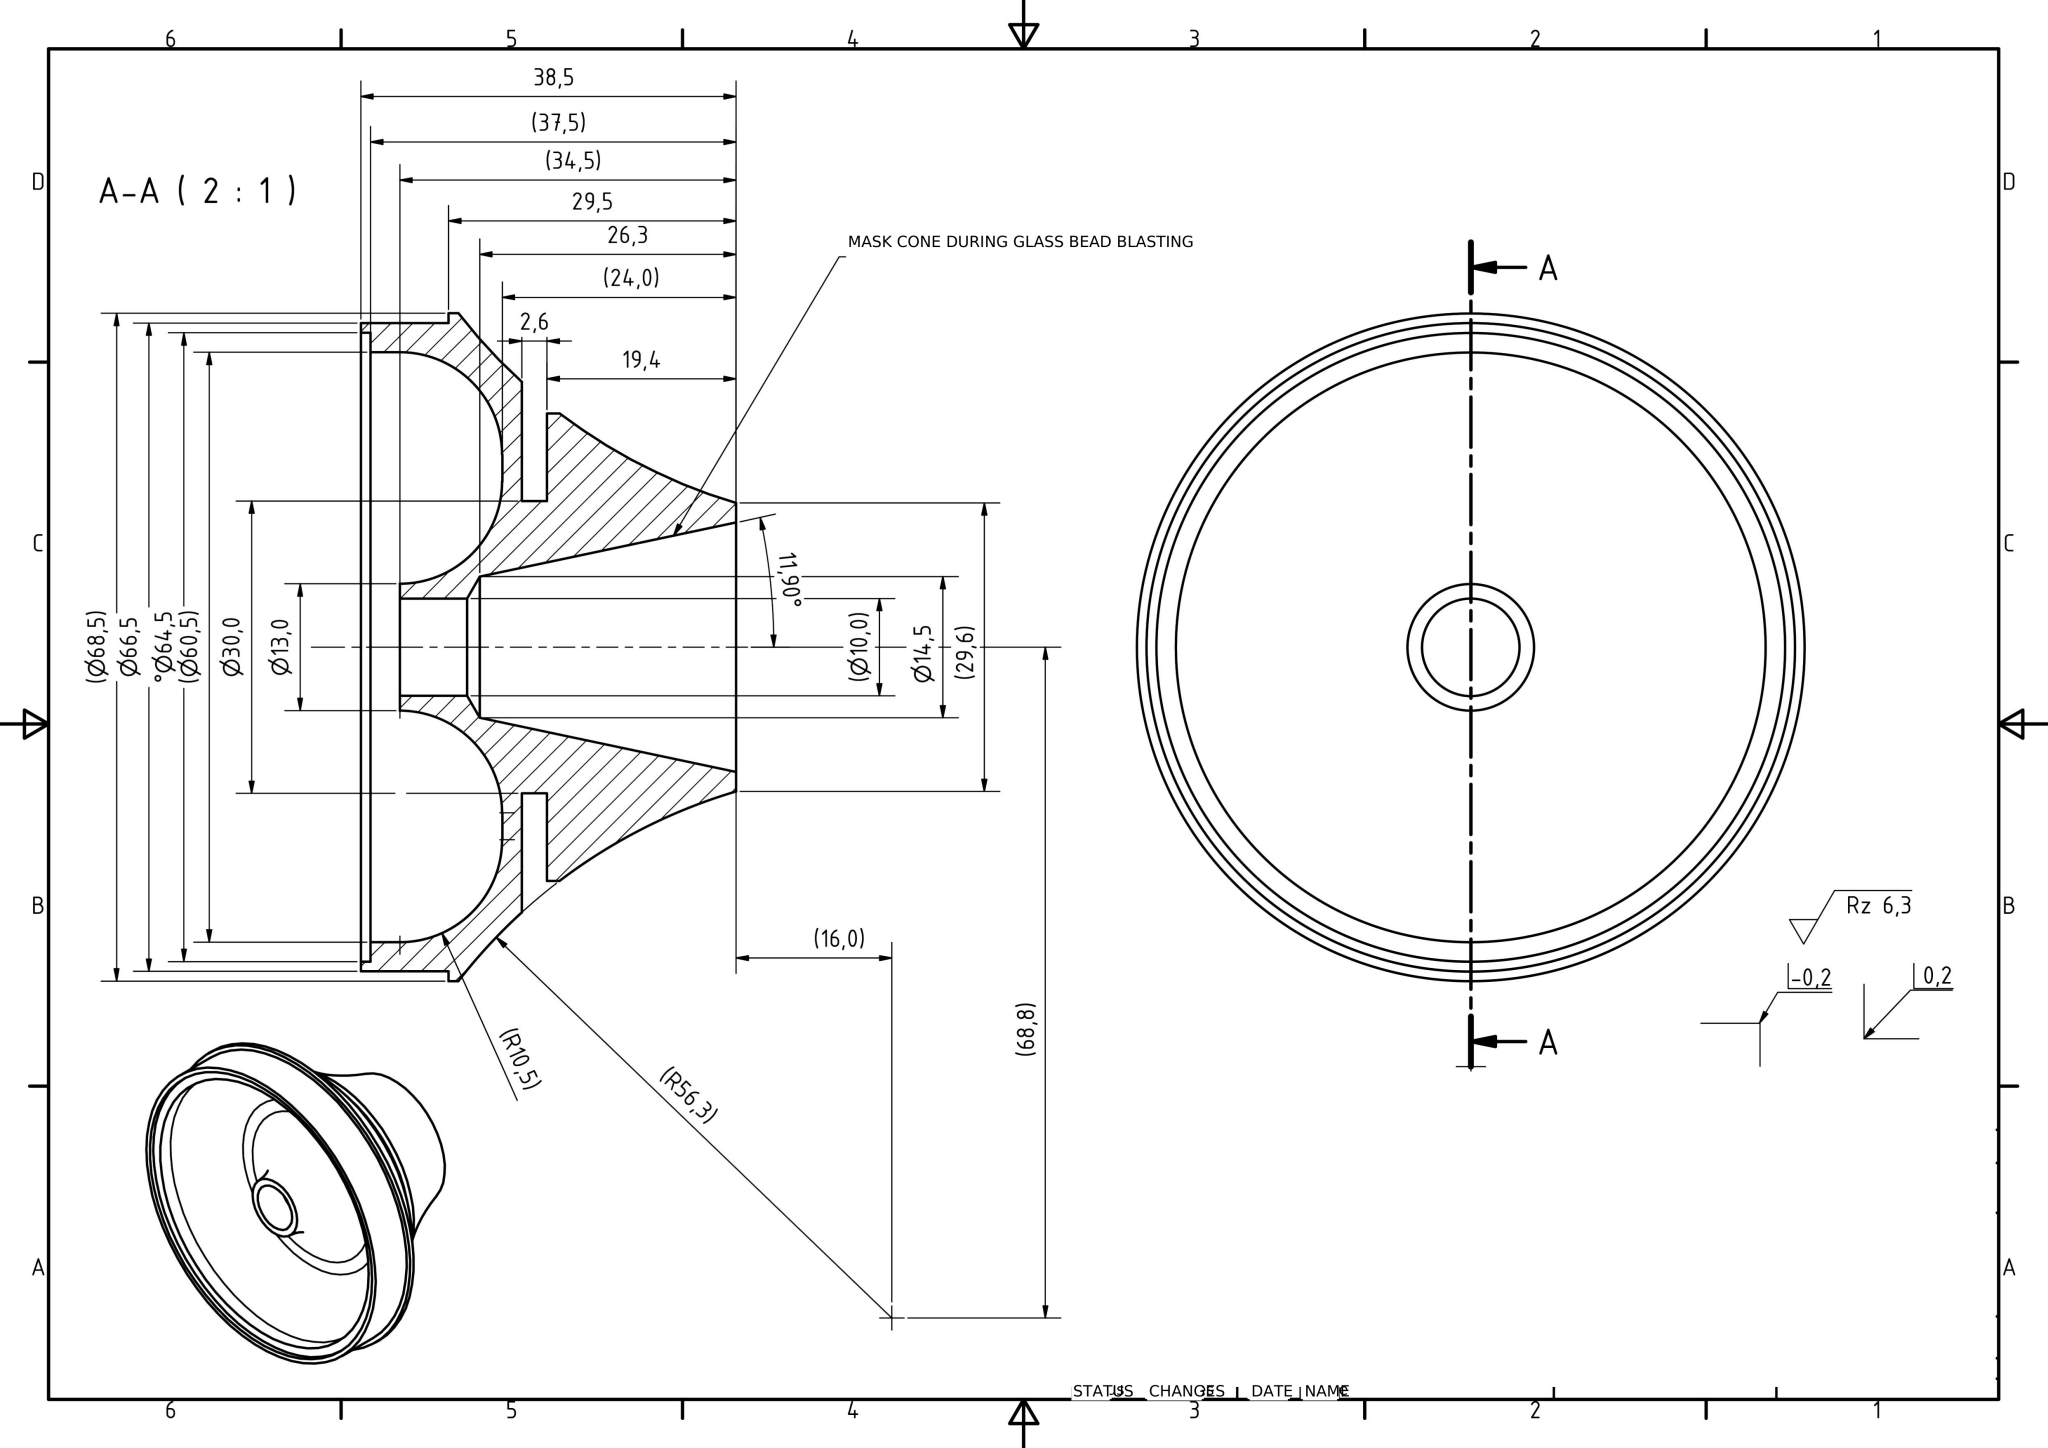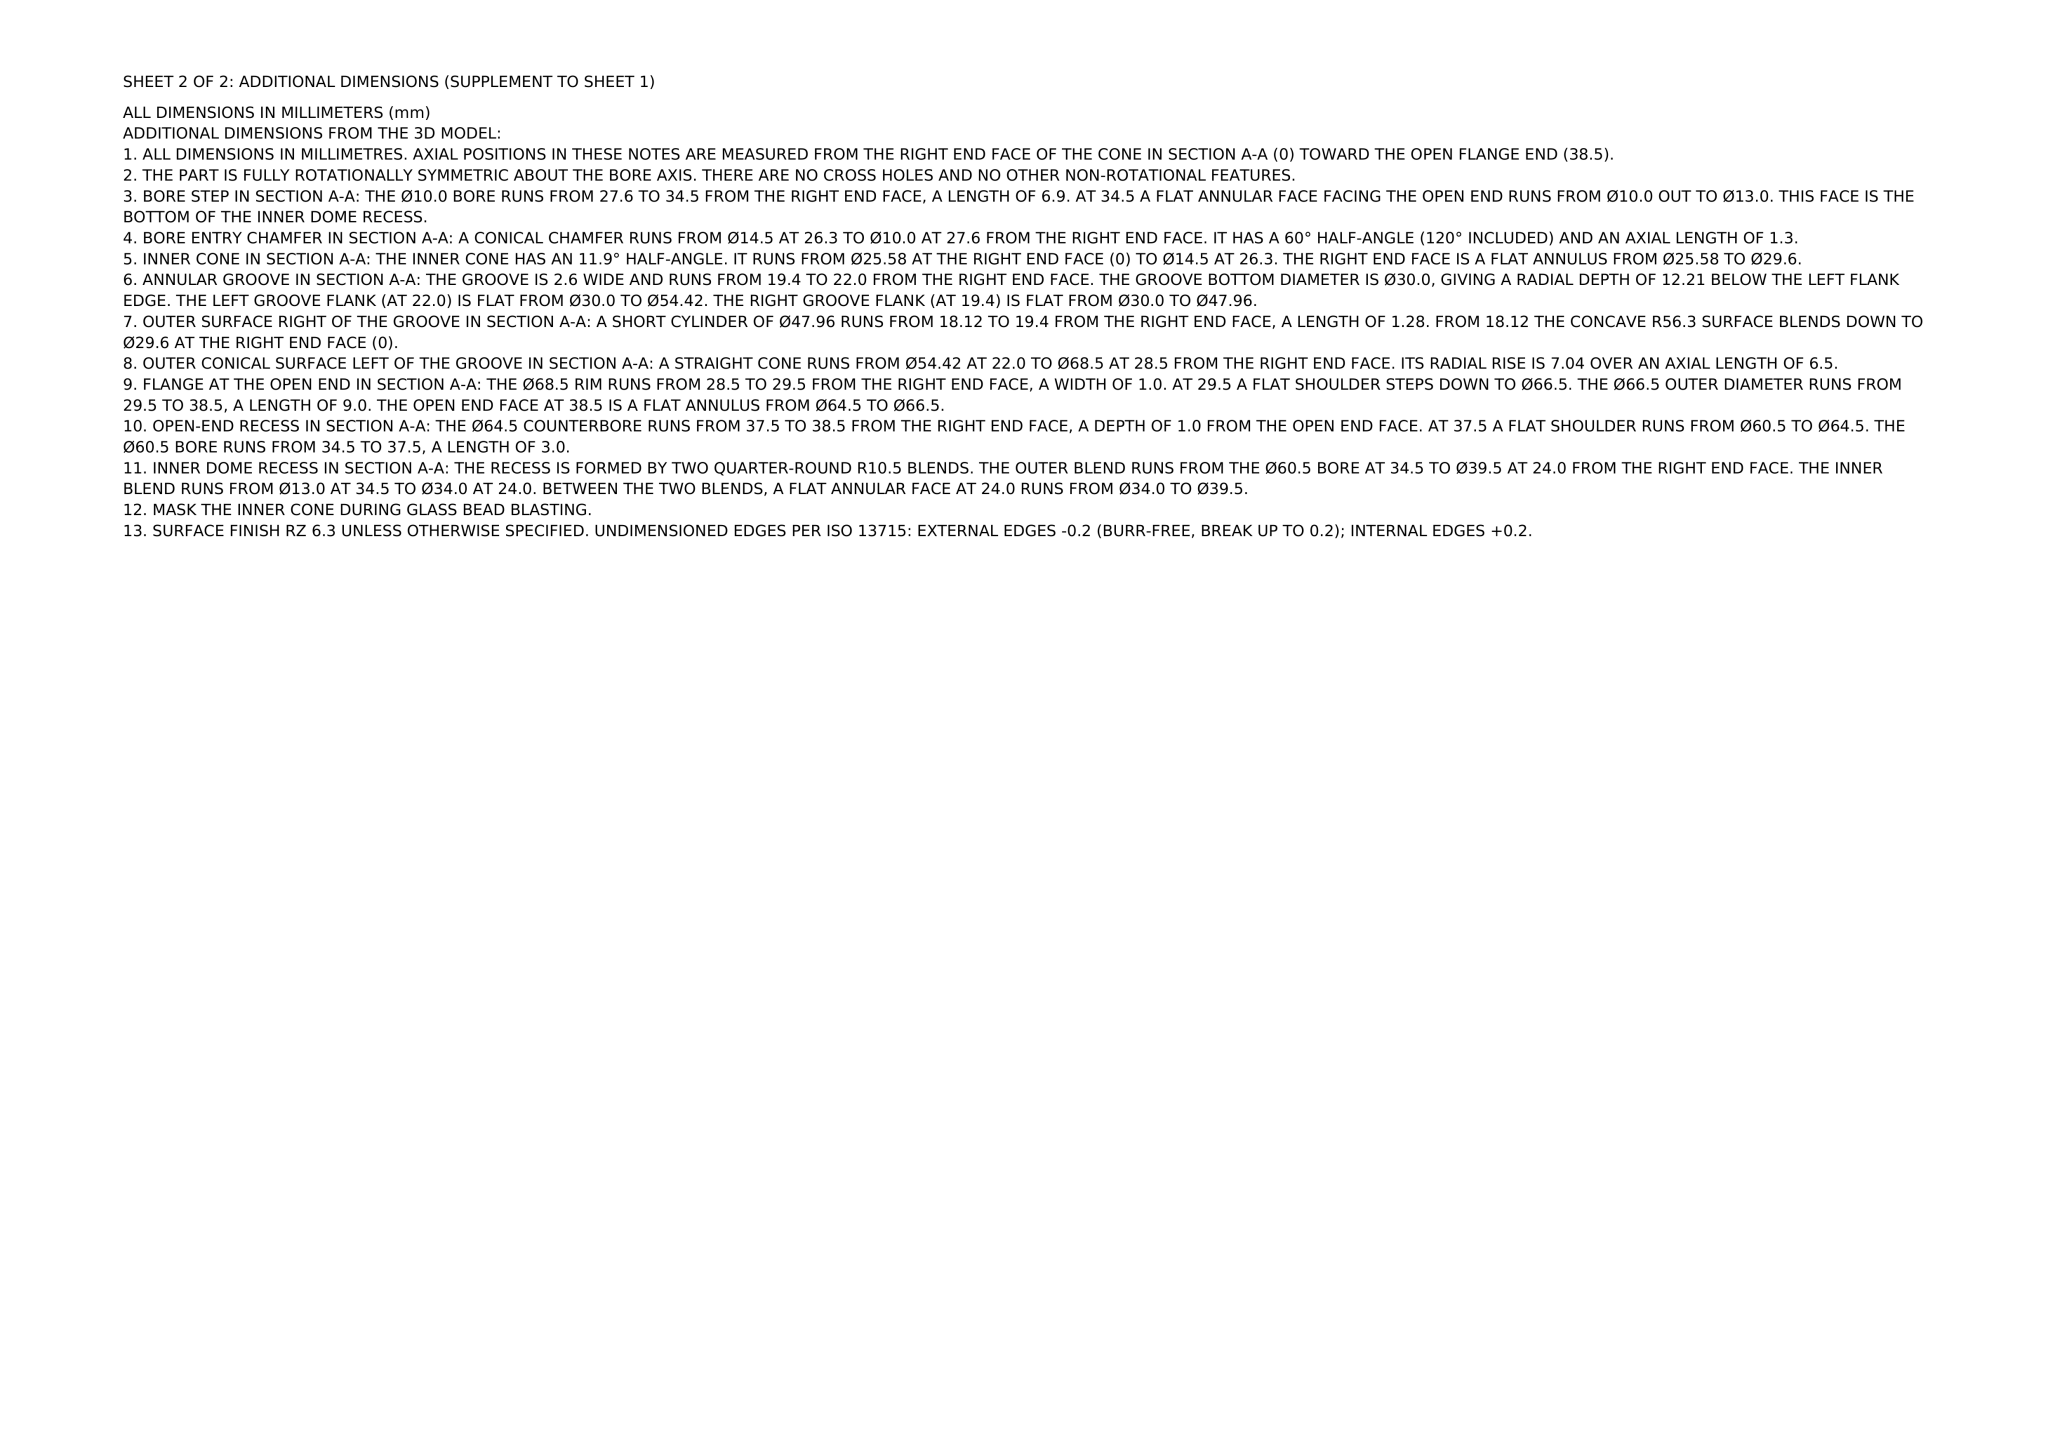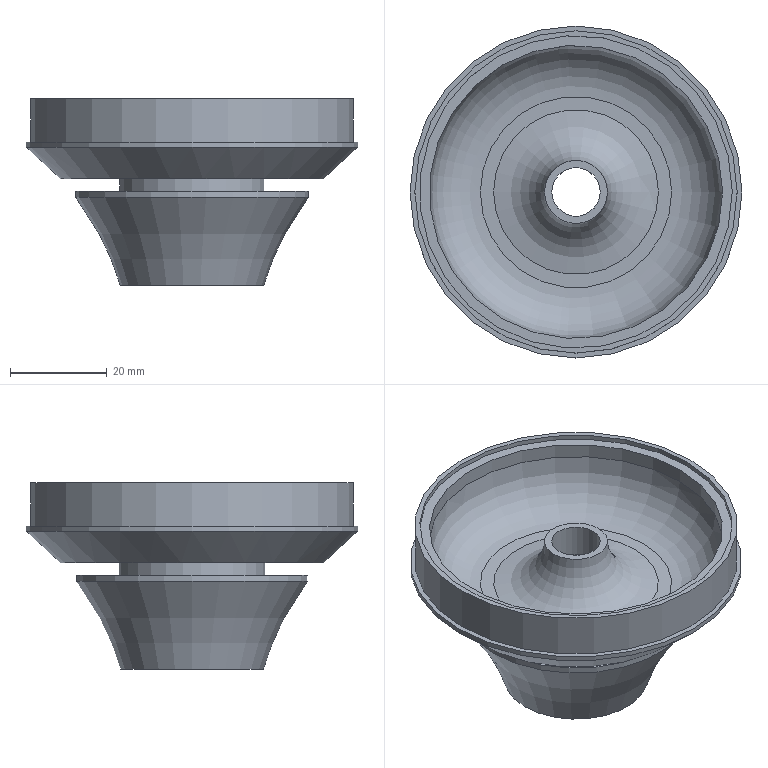Part | NX | mm | 1 solid | 21 faces | box 68.5 x 68.5 x 38.5 mm | volume 34087 mm3 | plane 8 | cylinder 7 | torus 4 | cone 2 | commonest cylinder face diameters 47.961 x1 30 x1 68.5 x1 66.5 x1 64.5 x1 60.5 x1 10 x1
STEP:
#1=COLOUR_RGB('',0.957,0.957,0.957);
#2=FILL_AREA_STYLE_COLOUR('',#1);
#3=FILL_AREA_STYLE('',(#2));
#4=SURFACE_STYLE_FILL_AREA(#3);
#5=SURFACE_SIDE_STYLE('',(#4));
#6=SURFACE_STYLE_USAGE(.BOTH.,#5);
#7=PRESENTATION_STYLE_ASSIGNMENT((#6));
#8=CARTESIAN_POINT('',(-23.98,0.,19.4));
#9=VERTEX_POINT('',#8);
#10=CARTESIAN_POINT('',(0.,0.,19.4));
#11=DIRECTION('',(0.,0.,1.));
#12=DIRECTION('',(-1.,0.,0.));
#13=AXIS2_PLACEMENT_3D('',#10,#11,#12);
#14=CIRCLE('',#13,23.98);
#15=EDGE_CURVE('',#9,#9,#14,.T.);
#16=ORIENTED_EDGE('',*,*,#15,.T.);
#17=EDGE_LOOP('',(#16));
#18=FACE_OUTER_BOUND('',#17,.T.);
#19=CARTESIAN_POINT('',(0.,15.,19.4));
#20=VERTEX_POINT('',#19);
#21=CARTESIAN_POINT('',(0.,0.,19.4));
#22=DIRECTION('',(0.,0.,-1.));
#23=DIRECTION('',(0.,1.,0.));
#24=AXIS2_PLACEMENT_3D('',#21,#22,#23);
#25=CIRCLE('',#24,15.);
#26=EDGE_CURVE('',#20,#20,#25,.T.);
#27=ORIENTED_EDGE('',*,*,#26,.T.);
#28=EDGE_LOOP('',(#27));
#29=FACE_BOUND('',#28,.T.);
#30=CARTESIAN_POINT('',(0.,19.99,19.4));
#31=DIRECTION('',(0.,0.,-1.));
#32=DIRECTION('',(-1.,0.,0.));
#33=AXIS2_PLACEMENT_3D('',#30,#31,#32);
#34=PLANE('',#33);
#35=ADVANCED_FACE('',(#18,#29),#34,.F.);
#36=STYLED_ITEM('',(#7),#35);
#37=CARTESIAN_POINT('',(0.,15.,22.));
#38=VERTEX_POINT('',#37);
#39=CARTESIAN_POINT('',(0.,0.,22.));
#40=DIRECTION('',(0.,0.,-1.));
#41=DIRECTION('',(0.,1.,0.));
#42=AXIS2_PLACEMENT_3D('',#39,#40,#41);
#43=CIRCLE('',#42,15.);
#44=EDGE_CURVE('',#38,#38,#43,.T.);
#45=ORIENTED_EDGE('',*,*,#44,.T.);
#46=EDGE_LOOP('',(#45));
#47=FACE_OUTER_BOUND('',#46,.T.);
#48=ORIENTED_EDGE('',*,*,#26,.F.);
#49=EDGE_LOOP('',(#48));
#50=FACE_BOUND('',#49,.T.);
#51=CARTESIAN_POINT('',(0.,0.,20.7));
#52=DIRECTION('',(0.,0.,-1.));
#53=DIRECTION('',(0.,1.,0.));
#54=AXIS2_PLACEMENT_3D('',#51,#52,#53);
#55=CYLINDRICAL_SURFACE('',#54,15.);
#56=ADVANCED_FACE('',(#47,#50),#55,.T.);
#57=STYLED_ITEM('',(#7),#56);
#58=CARTESIAN_POINT('',(0.,27.213,22.));
#59=VERTEX_POINT('',#58);
#60=CARTESIAN_POINT('',(0.,0.,22.));
#61=DIRECTION('',(0.,0.,1.));
#62=DIRECTION('',(0.,1.,0.));
#63=AXIS2_PLACEMENT_3D('',#60,#61,#62);
#64=CIRCLE('',#63,27.213);
#65=EDGE_CURVE('',#59,#59,#64,.T.);
#66=ORIENTED_EDGE('',*,*,#65,.F.);
#67=EDGE_LOOP('',(#66));
#68=FACE_OUTER_BOUND('',#67,.T.);
#69=ORIENTED_EDGE('',*,*,#44,.F.);
#70=EDGE_LOOP('',(#69));
#71=FACE_BOUND('',#70,.T.);
#72=CARTESIAN_POINT('',(0.,21.106,22.));
#73=DIRECTION('',(0.,0.,1.));
#74=DIRECTION('',(1.,0.,0.));
#75=AXIS2_PLACEMENT_3D('',#72,#73,#74);
#76=PLANE('',#75);
#77=ADVANCED_FACE('',(#68,#71),#76,.F.);
#78=STYLED_ITEM('',(#7),#77);
#79=CARTESIAN_POINT('',(34.25,0.,28.5));
#80=VERTEX_POINT('',#79);
#81=CARTESIAN_POINT('',(0.,0.,28.5));
#82=DIRECTION('',(0.,0.,1.));
#83=DIRECTION('',(1.,0.,0.));
#84=AXIS2_PLACEMENT_3D('',#81,#82,#83);
#85=CIRCLE('',#84,34.25);
#86=EDGE_CURVE('',#80,#80,#85,.T.);
#87=ORIENTED_EDGE('',*,*,#86,.F.);
#88=EDGE_LOOP('',(#87));
#89=FACE_OUTER_BOUND('',#88,.T.);
#90=ORIENTED_EDGE('',*,*,#65,.T.);
#91=EDGE_LOOP('',(#90));
#92=FACE_BOUND('',#91,.T.);
#93=CARTESIAN_POINT('',(0.,0.,-15.966));
#94=DIRECTION('',(0.,0.,1.));
#95=DIRECTION('',(1.,0.,0.));
#96=AXIS2_PLACEMENT_3D('',#93,#94,#95);
#97=TOROIDAL_SURFACE('',#96,68.8,56.311);
#98=ADVANCED_FACE('',(#89,#92),#97,.F.);
#99=STYLED_ITEM('',(#7),#98);
#100=CARTESIAN_POINT('',(23.98,-0.,18.124));
#101=VERTEX_POINT('',#100);
#102=CARTESIAN_POINT('',(0.,0.,18.124));
#103=DIRECTION('',(0.,0.,-1.));
#104=DIRECTION('',(-1.,0.,0.));
#105=AXIS2_PLACEMENT_3D('',#102,#103,#104);
#106=CIRCLE('',#105,23.98);
#107=EDGE_CURVE('',#101,#101,#106,.T.);
#108=ORIENTED_EDGE('',*,*,#107,.T.);
#109=EDGE_LOOP('',(#108));
#110=FACE_OUTER_BOUND('',#109,.T.);
#111=CARTESIAN_POINT('',(14.8,0.,0.));
#112=VERTEX_POINT('',#111);
#113=CARTESIAN_POINT('',(0.,0.,0.));
#114=DIRECTION('',(0.,0.,1.));
#115=DIRECTION('',(1.,0.,0.));
#116=AXIS2_PLACEMENT_3D('',#113,#114,#115);
#117=CIRCLE('',#116,14.8);
#118=EDGE_CURVE('',#112,#112,#117,.T.);
#119=ORIENTED_EDGE('',*,*,#118,.T.);
#120=EDGE_LOOP('',(#119));
#121=FACE_BOUND('',#120,.T.);
#122=CARTESIAN_POINT('',(0.,0.,-15.966));
#123=DIRECTION('',(0.,0.,1.));
#124=DIRECTION('',(1.,0.,0.));
#125=AXIS2_PLACEMENT_3D('',#122,#123,#124);
#126=TOROIDAL_SURFACE('',#125,68.8,56.311);
#127=ADVANCED_FACE('',(#110,#121),#126,.F.);
#128=STYLED_ITEM('',(#7),#127);
#129=CARTESIAN_POINT('',(34.25,0.,29.5));
#130=VERTEX_POINT('',#129);
#131=CARTESIAN_POINT('',(0.,0.,29.5));
#132=DIRECTION('',(0.,0.,1.));
#133=DIRECTION('',(1.,0.,0.));
#134=AXIS2_PLACEMENT_3D('',#131,#132,#133);
#135=CIRCLE('',#134,34.25);
#136=EDGE_CURVE('',#130,#130,#135,.T.);
#137=ORIENTED_EDGE('',*,*,#136,.F.);
#138=EDGE_LOOP('',(#137));
#139=FACE_OUTER_BOUND('',#138,.T.);
#140=ORIENTED_EDGE('',*,*,#86,.T.);
#141=EDGE_LOOP('',(#140));
#142=FACE_BOUND('',#141,.T.);
#143=CARTESIAN_POINT('',(0.,0.,29.));
#144=DIRECTION('',(0.,0.,1.));
#145=DIRECTION('',(1.,0.,0.));
#146=AXIS2_PLACEMENT_3D('',#143,#144,#145);
#147=CYLINDRICAL_SURFACE('',#146,34.25);
#148=ADVANCED_FACE('',(#139,#142),#147,.T.);
#149=STYLED_ITEM('',(#7),#148);
#150=ORIENTED_EDGE('',*,*,#136,.T.);
#151=EDGE_LOOP('',(#150));
#152=FACE_OUTER_BOUND('',#151,.T.);
#153=CARTESIAN_POINT('',(33.25,0.,29.5));
#154=VERTEX_POINT('',#153);
#155=CARTESIAN_POINT('',(0.,0.,29.5));
#156=DIRECTION('',(0.,0.,1.));
#157=DIRECTION('',(1.,0.,0.));
#158=AXIS2_PLACEMENT_3D('',#155,#156,#157);
#159=CIRCLE('',#158,33.25);
#160=EDGE_CURVE('',#154,#154,#159,.T.);
#161=ORIENTED_EDGE('',*,*,#160,.F.);
#162=EDGE_LOOP('',(#161));
#163=FACE_BOUND('',#162,.T.);
#164=CARTESIAN_POINT('',(33.75,0.,29.5));
#165=DIRECTION('',(0.,0.,1.));
#166=DIRECTION('',(1.,0.,0.));
#167=AXIS2_PLACEMENT_3D('',#164,#165,#166);
#168=PLANE('',#167);
#169=ADVANCED_FACE('',(#152,#163),#168,.T.);
#170=STYLED_ITEM('',(#7),#169);
#171=CARTESIAN_POINT('',(33.25,0.,38.5));
#172=VERTEX_POINT('',#171);
#173=CARTESIAN_POINT('',(0.,0.,38.5));
#174=DIRECTION('',(0.,0.,1.));
#175=DIRECTION('',(1.,0.,0.));
#176=AXIS2_PLACEMENT_3D('',#173,#174,#175);
#177=CIRCLE('',#176,33.25);
#178=EDGE_CURVE('',#172,#172,#177,.T.);
#179=ORIENTED_EDGE('',*,*,#178,.F.);
#180=EDGE_LOOP('',(#179));
#181=FACE_OUTER_BOUND('',#180,.T.);
#182=ORIENTED_EDGE('',*,*,#160,.T.);
#183=EDGE_LOOP('',(#182));
#184=FACE_BOUND('',#183,.T.);
#185=CARTESIAN_POINT('',(0.,0.,34.));
#186=DIRECTION('',(0.,0.,1.));
#187=DIRECTION('',(1.,0.,0.));
#188=AXIS2_PLACEMENT_3D('',#185,#186,#187);
#189=CYLINDRICAL_SURFACE('',#188,33.25);
#190=ADVANCED_FACE('',(#181,#184),#189,.T.);
#191=STYLED_ITEM('',(#7),#190);
#192=ORIENTED_EDGE('',*,*,#178,.T.);
#193=EDGE_LOOP('',(#192));
#194=FACE_OUTER_BOUND('',#193,.T.);
#195=CARTESIAN_POINT('',(32.25,0.,38.5));
#196=VERTEX_POINT('',#195);
#197=CARTESIAN_POINT('',(0.,0.,38.5));
#198=DIRECTION('',(0.,0.,1.));
#199=DIRECTION('',(1.,0.,0.));
#200=AXIS2_PLACEMENT_3D('',#197,#198,#199);
#201=CIRCLE('',#200,32.25);
#202=EDGE_CURVE('',#196,#196,#201,.T.);
#203=ORIENTED_EDGE('',*,*,#202,.F.);
#204=EDGE_LOOP('',(#203));
#205=FACE_BOUND('',#204,.T.);
#206=CARTESIAN_POINT('',(32.75,0.,38.5));
#207=DIRECTION('',(0.,0.,1.));
#208=DIRECTION('',(1.,0.,0.));
#209=AXIS2_PLACEMENT_3D('',#206,#207,#208);
#210=PLANE('',#209);
#211=ADVANCED_FACE('',(#194,#205),#210,.T.);
#212=STYLED_ITEM('',(#7),#211);
#213=CARTESIAN_POINT('',(32.25,0.,37.5));
#214=VERTEX_POINT('',#213);
#215=CARTESIAN_POINT('',(0.,0.,37.5));
#216=DIRECTION('',(0.,0.,1.));
#217=DIRECTION('',(1.,0.,0.));
#218=AXIS2_PLACEMENT_3D('',#215,#216,#217);
#219=CIRCLE('',#218,32.25);
#220=EDGE_CURVE('',#214,#214,#219,.T.);
#221=ORIENTED_EDGE('',*,*,#220,.F.);
#222=EDGE_LOOP('',(#221));
#223=FACE_OUTER_BOUND('',#222,.T.);
#224=ORIENTED_EDGE('',*,*,#202,.T.);
#225=EDGE_LOOP('',(#224));
#226=FACE_BOUND('',#225,.T.);
#227=CARTESIAN_POINT('',(0.,0.,38.));
#228=DIRECTION('',(0.,0.,1.));
#229=DIRECTION('',(1.,0.,0.));
#230=AXIS2_PLACEMENT_3D('',#227,#228,#229);
#231=CYLINDRICAL_SURFACE('',#230,32.25);
#232=ADVANCED_FACE('',(#223,#226),#231,.F.);
#233=STYLED_ITEM('',(#7),#232);
#234=ORIENTED_EDGE('',*,*,#220,.T.);
#235=EDGE_LOOP('',(#234));
#236=FACE_OUTER_BOUND('',#235,.T.);
#237=CARTESIAN_POINT('',(30.25,0.,37.5));
#238=VERTEX_POINT('',#237);
#239=CARTESIAN_POINT('',(0.,0.,37.5));
#240=DIRECTION('',(0.,0.,1.));
#241=DIRECTION('',(1.,0.,0.));
#242=AXIS2_PLACEMENT_3D('',#239,#240,#241);
#243=CIRCLE('',#242,30.25);
#244=EDGE_CURVE('',#238,#238,#243,.T.);
#245=ORIENTED_EDGE('',*,*,#244,.F.);
#246=EDGE_LOOP('',(#245));
#247=FACE_BOUND('',#246,.T.);
#248=CARTESIAN_POINT('',(31.25,0.,37.5));
#249=DIRECTION('',(0.,0.,1.));
#250=DIRECTION('',(1.,0.,0.));
#251=AXIS2_PLACEMENT_3D('',#248,#249,#250);
#252=PLANE('',#251);
#253=ADVANCED_FACE('',(#236,#247),#252,.T.);
#254=STYLED_ITEM('',(#7),#253);
#255=CARTESIAN_POINT('',(30.25,0.,34.5));
#256=VERTEX_POINT('',#255);
#257=CARTESIAN_POINT('',(0.,0.,34.5));
#258=DIRECTION('',(0.,0.,1.));
#259=DIRECTION('',(1.,0.,0.));
#260=AXIS2_PLACEMENT_3D('',#257,#258,#259);
#261=CIRCLE('',#260,30.25);
#262=EDGE_CURVE('',#256,#256,#261,.T.);
#263=ORIENTED_EDGE('',*,*,#262,.F.);
#264=EDGE_LOOP('',(#263));
#265=FACE_OUTER_BOUND('',#264,.T.);
#266=ORIENTED_EDGE('',*,*,#244,.T.);
#267=EDGE_LOOP('',(#266));
#268=FACE_BOUND('',#267,.T.);
#269=CARTESIAN_POINT('',(0.,0.,36.));
#270=DIRECTION('',(0.,0.,1.));
#271=DIRECTION('',(1.,0.,0.));
#272=AXIS2_PLACEMENT_3D('',#269,#270,#271);
#273=CYLINDRICAL_SURFACE('',#272,30.25);
#274=ADVANCED_FACE('',(#265,#268),#273,.F.);
#275=STYLED_ITEM('',(#7),#274);
#276=CARTESIAN_POINT('',(19.75,0.,24.));
#277=VERTEX_POINT('',#276);
#278=CARTESIAN_POINT('',(0.,0.,24.));
#279=DIRECTION('',(0.,0.,1.));
#280=DIRECTION('',(1.,0.,0.));
#281=AXIS2_PLACEMENT_3D('',#278,#279,#280);
#282=CIRCLE('',#281,19.75);
#283=EDGE_CURVE('',#277,#277,#282,.T.);
#284=ORIENTED_EDGE('',*,*,#283,.F.);
#285=EDGE_LOOP('',(#284));
#286=FACE_OUTER_BOUND('',#285,.T.);
#287=ORIENTED_EDGE('',*,*,#262,.T.);
#288=EDGE_LOOP('',(#287));
#289=FACE_BOUND('',#288,.T.);
#290=CARTESIAN_POINT('',(0.,0.,34.5));
#291=DIRECTION('',(0.,0.,1.));
#292=DIRECTION('',(1.,0.,0.));
#293=AXIS2_PLACEMENT_3D('',#290,#291,#292);
#294=TOROIDAL_SURFACE('',#293,19.75,10.5);
#295=ADVANCED_FACE('',(#286,#289),#294,.F.);
#296=STYLED_ITEM('',(#7),#295);
#297=ORIENTED_EDGE('',*,*,#283,.T.);
#298=EDGE_LOOP('',(#297));
#299=FACE_OUTER_BOUND('',#298,.T.);
#300=CARTESIAN_POINT('',(17.,0.,24.));
#301=VERTEX_POINT('',#300);
#302=CARTESIAN_POINT('',(0.,0.,24.));
#303=DIRECTION('',(0.,0.,1.));
#304=DIRECTION('',(1.,0.,0.));
#305=AXIS2_PLACEMENT_3D('',#302,#303,#304);
#306=CIRCLE('',#305,17.);
#307=EDGE_CURVE('',#301,#301,#306,.T.);
#308=ORIENTED_EDGE('',*,*,#307,.F.);
#309=EDGE_LOOP('',(#308));
#310=FACE_BOUND('',#309,.T.);
#311=CARTESIAN_POINT('',(18.375,0.,24.));
#312=DIRECTION('',(0.,0.,1.));
#313=DIRECTION('',(1.,0.,0.));
#314=AXIS2_PLACEMENT_3D('',#311,#312,#313);
#315=PLANE('',#314);
#316=ADVANCED_FACE('',(#299,#310),#315,.T.);
#317=STYLED_ITEM('',(#7),#316);
#318=CARTESIAN_POINT('',(6.5,0.,34.5));
#319=VERTEX_POINT('',#318);
#320=CARTESIAN_POINT('',(0.,0.,34.5));
#321=DIRECTION('',(0.,0.,1.));
#322=DIRECTION('',(1.,0.,0.));
#323=AXIS2_PLACEMENT_3D('',#320,#321,#322);
#324=CIRCLE('',#323,6.5);
#325=EDGE_CURVE('',#319,#319,#324,.T.);
#326=ORIENTED_EDGE('',*,*,#325,.F.);
#327=EDGE_LOOP('',(#326));
#328=FACE_OUTER_BOUND('',#327,.T.);
#329=ORIENTED_EDGE('',*,*,#307,.T.);
#330=EDGE_LOOP('',(#329));
#331=FACE_BOUND('',#330,.T.);
#332=CARTESIAN_POINT('',(0.,0.,34.5));
#333=DIRECTION('',(0.,0.,1.));
#334=DIRECTION('',(1.,0.,0.));
#335=AXIS2_PLACEMENT_3D('',#332,#333,#334);
#336=TOROIDAL_SURFACE('',#335,17.,10.5);
#337=ADVANCED_FACE('',(#328,#331),#336,.F.);
#338=STYLED_ITEM('',(#7),#337);
#339=ORIENTED_EDGE('',*,*,#325,.T.);
#340=EDGE_LOOP('',(#339));
#341=FACE_OUTER_BOUND('',#340,.T.);
#342=CARTESIAN_POINT('',(5.,0.,34.5));
#343=VERTEX_POINT('',#342);
#344=CARTESIAN_POINT('',(0.,0.,34.5));
#345=DIRECTION('',(0.,0.,1.));
#346=DIRECTION('',(1.,0.,0.));
#347=AXIS2_PLACEMENT_3D('',#344,#345,#346);
#348=CIRCLE('',#347,5.);
#349=EDGE_CURVE('',#343,#343,#348,.T.);
#350=ORIENTED_EDGE('',*,*,#349,.F.);
#351=EDGE_LOOP('',(#350));
#352=FACE_BOUND('',#351,.T.);
#353=CARTESIAN_POINT('',(5.75,0.,34.5));
#354=DIRECTION('',(0.,0.,1.));
#355=DIRECTION('',(1.,0.,0.));
#356=AXIS2_PLACEMENT_3D('',#353,#354,#355);
#357=PLANE('',#356);
#358=ADVANCED_FACE('',(#341,#352),#357,.T.);
#359=STYLED_ITEM('',(#7),#358);
#360=CARTESIAN_POINT('',(5.,0.,27.599));
#361=VERTEX_POINT('',#360);
#362=CARTESIAN_POINT('',(0.,0.,27.599));
#363=DIRECTION('',(0.,0.,1.));
#364=DIRECTION('',(1.,0.,0.));
#365=AXIS2_PLACEMENT_3D('',#362,#363,#364);
#366=CIRCLE('',#365,5.);
#367=EDGE_CURVE('',#361,#361,#366,.T.);
#368=ORIENTED_EDGE('',*,*,#367,.F.);
#369=EDGE_LOOP('',(#368));
#370=FACE_OUTER_BOUND('',#369,.T.);
#371=ORIENTED_EDGE('',*,*,#349,.T.);
#372=EDGE_LOOP('',(#371));
#373=FACE_BOUND('',#372,.T.);
#374=CARTESIAN_POINT('',(0.,0.,31.05));
#375=DIRECTION('',(0.,0.,1.));
#376=DIRECTION('',(1.,0.,0.));
#377=AXIS2_PLACEMENT_3D('',#374,#375,#376);
#378=CYLINDRICAL_SURFACE('',#377,5.);
#379=ADVANCED_FACE('',(#370,#373),#378,.F.);
#380=STYLED_ITEM('',(#7),#379);
#381=CARTESIAN_POINT('',(7.25,0.,26.3));
#382=VERTEX_POINT('',#381);
#383=CARTESIAN_POINT('',(0.,0.,26.3));
#384=DIRECTION('',(0.,0.,1.));
#385=DIRECTION('',(1.,0.,0.));
#386=AXIS2_PLACEMENT_3D('',#383,#384,#385);
#387=CIRCLE('',#386,7.25);
#388=EDGE_CURVE('',#382,#382,#387,.T.);
#389=ORIENTED_EDGE('',*,*,#388,.F.);
#390=EDGE_LOOP('',(#389));
#391=FACE_OUTER_BOUND('',#390,.T.);
#392=ORIENTED_EDGE('',*,*,#367,.T.);
#393=EDGE_LOOP('',(#392));
#394=FACE_BOUND('',#393,.T.);
#395=CARTESIAN_POINT('',(0.,0.,26.95));
#396=DIRECTION('',(0.,0.,-1.));
#397=DIRECTION('',(1.,0.,0.));
#398=AXIS2_PLACEMENT_3D('',#395,#396,#397);
#399=CONICAL_SURFACE('',#398,6.125,60.);
#400=ADVANCED_FACE('',(#391,#394),#399,.F.);
#401=STYLED_ITEM('',(#7),#400);
#402=CARTESIAN_POINT('',(12.792,0.,-0.));
#403=VERTEX_POINT('',#402);
#404=CARTESIAN_POINT('',(0.,0.,-0.));
#405=DIRECTION('',(0.,0.,1.));
#406=DIRECTION('',(1.,0.,0.));
#407=AXIS2_PLACEMENT_3D('',#404,#405,#406);
#408=CIRCLE('',#407,12.792);
#409=EDGE_CURVE('',#403,#403,#408,.T.);
#410=ORIENTED_EDGE('',*,*,#409,.F.);
#411=EDGE_LOOP('',(#410));
#412=FACE_OUTER_BOUND('',#411,.T.);
#413=ORIENTED_EDGE('',*,*,#388,.T.);
#414=EDGE_LOOP('',(#413));
#415=FACE_BOUND('',#414,.T.);
#416=CARTESIAN_POINT('',(0.,0.,13.15));
#417=DIRECTION('',(0.,0.,-1.));
#418=DIRECTION('',(1.,0.,0.));
#419=AXIS2_PLACEMENT_3D('',#416,#417,#418);
#420=CONICAL_SURFACE('',#419,10.021,11.9);
#421=ADVANCED_FACE('',(#412,#415),#420,.F.);
#422=STYLED_ITEM('',(#7),#421);
#423=ORIENTED_EDGE('',*,*,#118,.F.);
#424=EDGE_LOOP('',(#423));
#425=FACE_OUTER_BOUND('',#424,.T.);
#426=ORIENTED_EDGE('',*,*,#409,.T.);
#427=EDGE_LOOP('',(#426));
#428=FACE_BOUND('',#427,.T.);
#429=CARTESIAN_POINT('',(13.796,0.,-0.));
#430=DIRECTION('',(0.,0.,-1.));
#431=DIRECTION('',(-1.,0.,0.));
#432=AXIS2_PLACEMENT_3D('',#429,#430,#431);
#433=PLANE('',#432);
#434=ADVANCED_FACE('',(#425,#428),#433,.T.);
#435=STYLED_ITEM('',(#7),#434);
#436=COLOUR_RGB('',0.898,0.9,0.9);
#437=FILL_AREA_STYLE_COLOUR('',#436);
#438=FILL_AREA_STYLE('',(#437));
#439=SURFACE_STYLE_FILL_AREA(#438);
#440=SURFACE_SIDE_STYLE('',(#439));
#441=SURFACE_STYLE_USAGE(.BOTH.,#440);
#442=PRESENTATION_STYLE_ASSIGNMENT((#441));
#443=ORIENTED_EDGE('',*,*,#107,.F.);
#444=EDGE_LOOP('',(#443));
#445=FACE_OUTER_BOUND('',#444,.T.);
#446=ORIENTED_EDGE('',*,*,#15,.F.);
#447=EDGE_LOOP('',(#446));
#448=FACE_BOUND('',#447,.T.);
#449=CARTESIAN_POINT('',(0.,0.,16.925));
#450=DIRECTION('',(0.,0.,1.));
#451=DIRECTION('',(-1.,0.,0.));
#452=AXIS2_PLACEMENT_3D('',#449,#450,#451);
#453=CYLINDRICAL_SURFACE('',#452,23.98);
#454=ADVANCED_FACE('',(#445,#448),#453,.T.);
#455=CLOSED_SHELL('',(#454,#35,#56,#77,#98,#127,#148,#169,#190,#211,#232,#253,#274,#295,#316,#337,#358,#379,#400,#421,#434));
#456=MANIFOLD_SOLID_BREP('',#455);
#457=STYLED_ITEM('',(#442),#456);
#458=(LENGTH_UNIT()NAMED_UNIT(*)SI_UNIT(.MILLI.,.METRE.));
#459=UNCERTAINTY_MEASURE_WITH_UNIT(LENGTH_MEASURE(0.000001),#458,'','');
#460=(NAMED_UNIT(*)PLANE_ANGLE_UNIT()SI_UNIT($,.RADIAN.));
#461=PLANE_ANGLE_MEASURE_WITH_UNIT(PLANE_ANGLE_MEASURE(0.01745),#460);
#462=DIMENSIONAL_EXPONENTS(0.,0.,0.,0.,0.,0.,0.);
#463=(CONVERSION_BASED_UNIT('',#461)NAMED_UNIT(#462)PLANE_ANGLE_UNIT());
#464=(NAMED_UNIT(*)SI_UNIT($,.STERADIAN.)SOLID_ANGLE_UNIT());
#465=(GEOMETRIC_REPRESENTATION_CONTEXT(3)GLOBAL_UNCERTAINTY_ASSIGNED_CONTEXT((#459))GLOBAL_UNIT_ASSIGNED_CONTEXT((#463,#464,#458))REPRESENTATION_CONTEXT('',''));
#466=MECHANICAL_DESIGN_GEOMETRIC_PRESENTATION_REPRESENTATION('',(#36,#57,#78,#99,#128,#149,#170,#191,#212,#233,#254,#275,#296,#317,#338,#359,#380,#401,#422,#435,#457),#465);
#467=(LENGTH_UNIT()NAMED_UNIT(*)SI_UNIT(.MILLI.,.METRE.));
#468=UNCERTAINTY_MEASURE_WITH_UNIT(LENGTH_MEASURE(0.01),#467,'','');
#469=(NAMED_UNIT(*)PLANE_ANGLE_UNIT()SI_UNIT($,.RADIAN.));
#470=PLANE_ANGLE_MEASURE_WITH_UNIT(PLANE_ANGLE_MEASURE(0.01745),#469);
#471=DIMENSIONAL_EXPONENTS(0.,0.,0.,0.,0.,0.,0.);
#472=(CONVERSION_BASED_UNIT('',#470)NAMED_UNIT(#471)PLANE_ANGLE_UNIT());
#473=(NAMED_UNIT(*)SI_UNIT($,.STERADIAN.)SOLID_ANGLE_UNIT());
#474=(GEOMETRIC_REPRESENTATION_CONTEXT(3)GLOBAL_UNCERTAINTY_ASSIGNED_CONTEXT((#468))GLOBAL_UNIT_ASSIGNED_CONTEXT((#472,#473,#467))REPRESENTATION_CONTEXT('',''));
#475=ADVANCED_BREP_SHAPE_REPRESENTATION('',(#456),#474);
#476=CARTESIAN_POINT('',(0.,0.,0.));
#477=DIRECTION('',(0.,0.,1.));
#478=DIRECTION('',(1.,0.,0.));
#479=AXIS2_PLACEMENT_3D('',#476,#477,#478);
#480=SHAPE_REPRESENTATION('',(#479),#474);
#481=SHAPE_REPRESENTATION_RELATIONSHIP('','',#475,#480);